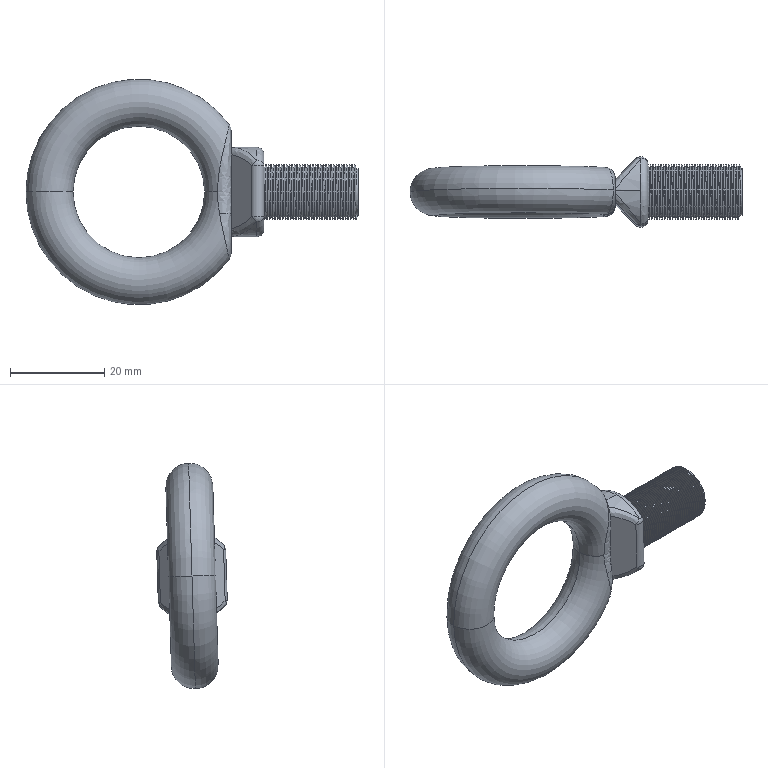Component | SolidWorks | M12LiftingEye-1 | 1 solid | 174 faces | volume 11932 mm3 | cylinder 149 | spline 8 | torus 7 | plane 6 | sphere 4 | commonest cylinder face diameters 10 x73 11.619 x71 19 x3 3 x2